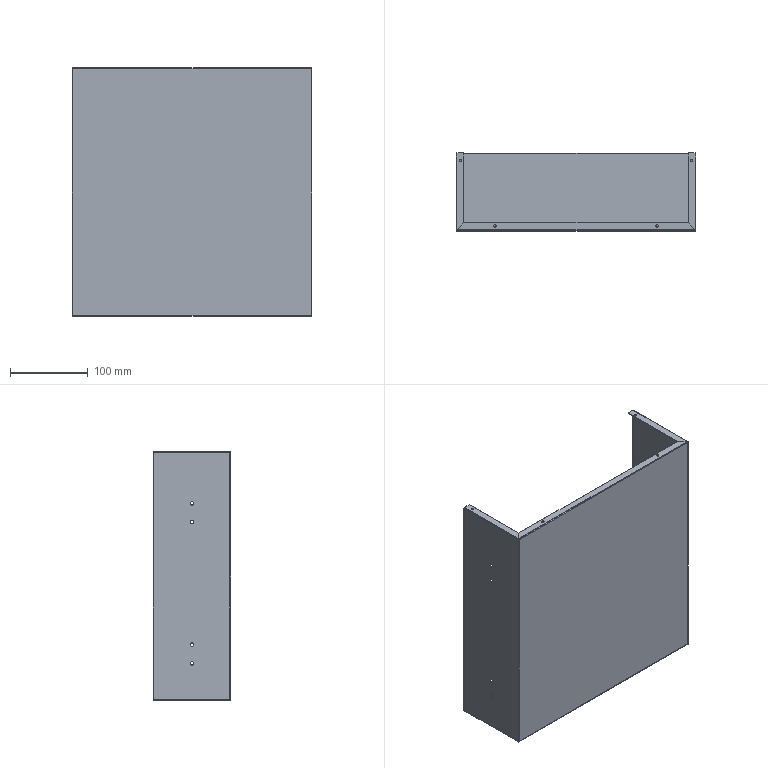Component | SolidWorks | DrawerWelding-1_Drawer-1 | 1 solid | 84 faces | volume 196464 mm3 | plane 44 | cylinder 36 | spline 4 | commonest cylinder face diameters 4.5 x16 3 x8 2.2 x6 0.2 x6